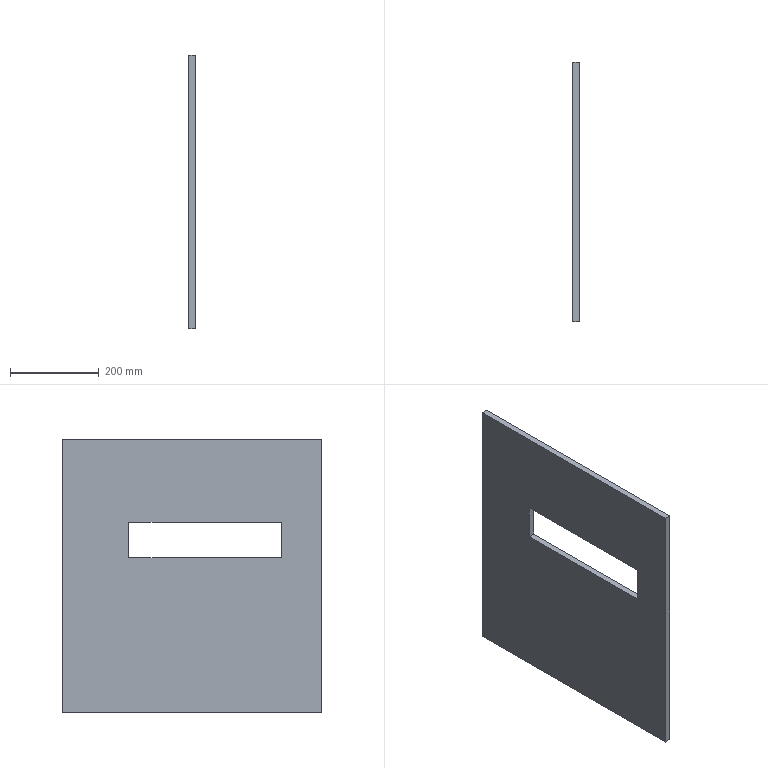Component | NX | PLATE | 1 solid | 10 faces | box 15 x 585 x 618 mm | volume 5008950 mm3 | plane 10
STEP:
#1=CARTESIAN_POINT('',(0.,0.,0.));
#2=DIRECTION('',(0.,0.,1.));
#3=DIRECTION('',(1.,0.,0.));
#4=AXIS2_PLACEMENT_3D('',#1,#2,#3);
#5=CARTESIAN_POINT('',(1548.254,590.,470.));
#6=VERTEX_POINT('',#5);
#7=CARTESIAN_POINT('',(1548.254,935.,470.));
#8=VERTEX_POINT('',#7);
#9=CARTESIAN_POINT('',(1548.254,935.,470.));
#10=DIRECTION('',(0.,1.,0.));
#11=VECTOR('',#10,1.);
#12=LINE('',#9,#11);
#13=CARTESIAN_POINT('',(1533.254,935.,470.));
#14=DIRECTION('',(0.,0.,1.));
#15=DIRECTION('',(0.,-1.,0.));
#16=AXIS2_PLACEMENT_3D('',#13,#14,#15);
#17=PLANE('',#16);
#18=CARTESIAN_POINT('',(0.,15.));
#19=DIRECTION('',(-1.,0.));
#20=VECTOR('',#19,1.);
#21=LINE('',#18,#20);
#22=(GEOMETRIC_REPRESENTATION_CONTEXT(2)PARAMETRIC_REPRESENTATION_CONTEXT()REPRESENTATION_CONTEXT('',''));
#23=DEFINITIONAL_REPRESENTATION('',(#21),#22);
#24=PCURVE('',#17,#23);
#25=CARTESIAN_POINT('',(1548.254,1295.392,39.213));
#26=DIRECTION('',(1.,0.,0.));
#27=DIRECTION('',(0.,1.,0.));
#28=AXIS2_PLACEMENT_3D('',#25,#26,#27);
#29=PLANE('',#28);
#30=CARTESIAN_POINT('',(-360.392,430.787));
#31=DIRECTION('',(1.,0.));
#32=VECTOR('',#31,1.);
#33=LINE('',#30,#32);
#34=(GEOMETRIC_REPRESENTATION_CONTEXT(2)PARAMETRIC_REPRESENTATION_CONTEXT()REPRESENTATION_CONTEXT('',''));
#35=DEFINITIONAL_REPRESENTATION('',(#33),#34);
#36=PCURVE('',#29,#35);
#37=SURFACE_CURVE('',#12,(#24,#36),.PCURVE_S1.);
#38=EDGE_CURVE('',#6,#8,#37,.T.);
#39=ORIENTED_EDGE('',*,*,#38,.T.);
#40=CARTESIAN_POINT('',(1533.254,935.,470.));
#41=VERTEX_POINT('',#40);
#42=CARTESIAN_POINT('',(1533.254,935.,470.));
#43=DIRECTION('',(-1.,0.,0.));
#44=VECTOR('',#43,1.);
#45=LINE('',#42,#44);
#46=CARTESIAN_POINT('',(0.,0.));
#47=DIRECTION('',(0.,-1.));
#48=VECTOR('',#47,1.);
#49=LINE('',#46,#48);
#50=(GEOMETRIC_REPRESENTATION_CONTEXT(2)PARAMETRIC_REPRESENTATION_CONTEXT()REPRESENTATION_CONTEXT('',''));
#51=DEFINITIONAL_REPRESENTATION('',(#49),#50);
#52=PCURVE('',#17,#51);
#53=CARTESIAN_POINT('',(1533.254,935.,550.));
#54=DIRECTION('',(0.,-1.,0.));
#55=DIRECTION('',(1.,0.,0.));
#56=AXIS2_PLACEMENT_3D('',#53,#54,#55);
#57=PLANE('',#56);
#58=CARTESIAN_POINT('',(0.,-80.));
#59=DIRECTION('',(-1.,0.));
#60=VECTOR('',#59,1.);
#61=LINE('',#58,#60);
#62=(GEOMETRIC_REPRESENTATION_CONTEXT(2)PARAMETRIC_REPRESENTATION_CONTEXT()REPRESENTATION_CONTEXT('',''));
#63=DEFINITIONAL_REPRESENTATION('',(#61),#62);
#64=PCURVE('',#57,#63);
#65=SURFACE_CURVE('',#45,(#52,#64),.PCURVE_S1.);
#66=EDGE_CURVE('',#8,#41,#65,.T.);
#67=ORIENTED_EDGE('',*,*,#66,.T.);
#68=CARTESIAN_POINT('',(1533.254,590.,470.));
#69=VERTEX_POINT('',#68);
#70=CARTESIAN_POINT('',(1533.254,935.,470.));
#71=DIRECTION('',(0.,1.,0.));
#72=VECTOR('',#71,1.);
#73=LINE('',#70,#72);
#74=CARTESIAN_POINT('',(0.,0.));
#75=DIRECTION('',(-1.,0.));
#76=VECTOR('',#75,1.);
#77=LINE('',#74,#76);
#78=(GEOMETRIC_REPRESENTATION_CONTEXT(2)PARAMETRIC_REPRESENTATION_CONTEXT()REPRESENTATION_CONTEXT('',''));
#79=DEFINITIONAL_REPRESENTATION('',(#77),#78);
#80=PCURVE('',#17,#79);
#81=CARTESIAN_POINT('',(1533.254,1295.392,39.213));
#82=DIRECTION('',(1.,0.,0.));
#83=DIRECTION('',(0.,1.,0.));
#84=AXIS2_PLACEMENT_3D('',#81,#82,#83);
#85=PLANE('',#84);
#86=CARTESIAN_POINT('',(-360.392,430.787));
#87=DIRECTION('',(1.,0.));
#88=VECTOR('',#87,1.);
#89=LINE('',#86,#88);
#90=(GEOMETRIC_REPRESENTATION_CONTEXT(2)PARAMETRIC_REPRESENTATION_CONTEXT()REPRESENTATION_CONTEXT('',''));
#91=DEFINITIONAL_REPRESENTATION('',(#89),#90);
#92=PCURVE('',#85,#91);
#93=SURFACE_CURVE('',#73,(#80,#92),.PCURVE_S1.);
#94=EDGE_CURVE('',#69,#41,#93,.T.);
#95=ORIENTED_EDGE('',*,*,#94,.F.);
#96=CARTESIAN_POINT('',(1533.254,590.,470.));
#97=DIRECTION('',(-1.,0.,0.));
#98=VECTOR('',#97,1.);
#99=LINE('',#96,#98);
#100=CARTESIAN_POINT('',(345.,0.));
#101=DIRECTION('',(0.,-1.));
#102=VECTOR('',#101,1.);
#103=LINE('',#100,#102);
#104=(GEOMETRIC_REPRESENTATION_CONTEXT(2)PARAMETRIC_REPRESENTATION_CONTEXT()REPRESENTATION_CONTEXT('',''));
#105=DEFINITIONAL_REPRESENTATION('',(#103),#104);
#106=PCURVE('',#17,#105);
#107=CARTESIAN_POINT('',(1533.254,590.,470.));
#108=DIRECTION('',(0.,1.,0.));
#109=DIRECTION('',(-1.,0.,0.));
#110=AXIS2_PLACEMENT_3D('',#107,#108,#109);
#111=PLANE('',#110);
#112=CARTESIAN_POINT('',(0.,0.));
#113=DIRECTION('',(1.,0.));
#114=VECTOR('',#113,1.);
#115=LINE('',#112,#114);
#116=(GEOMETRIC_REPRESENTATION_CONTEXT(2)PARAMETRIC_REPRESENTATION_CONTEXT()REPRESENTATION_CONTEXT('',''));
#117=DEFINITIONAL_REPRESENTATION('',(#115),#116);
#118=PCURVE('',#111,#117);
#119=SURFACE_CURVE('',#99,(#106,#118),.PCURVE_S1.);
#120=EDGE_CURVE('',#6,#69,#119,.T.);
#121=ORIENTED_EDGE('',*,*,#120,.F.);
#122=EDGE_LOOP('',(#39,#67,#95,#121));
#123=FACE_BOUND('',#122,.T.);
#124=ADVANCED_FACE('',(#123),#17,.T.);
#125=CARTESIAN_POINT('',(1548.254,590.,550.));
#126=VERTEX_POINT('',#125);
#127=CARTESIAN_POINT('',(1548.254,590.,470.));
#128=DIRECTION('',(0.,0.,-1.));
#129=VECTOR('',#128,1.);
#130=LINE('',#127,#129);
#131=CARTESIAN_POINT('',(-15.,0.));
#132=DIRECTION('',(0.,-1.));
#133=VECTOR('',#132,1.);
#134=LINE('',#131,#133);
#135=(GEOMETRIC_REPRESENTATION_CONTEXT(2)PARAMETRIC_REPRESENTATION_CONTEXT()REPRESENTATION_CONTEXT('',''));
#136=DEFINITIONAL_REPRESENTATION('',(#134),#135);
#137=PCURVE('',#111,#136);
#138=CARTESIAN_POINT('',(-705.392,430.787));
#139=DIRECTION('',(0.,-1.));
#140=VECTOR('',#139,1.);
#141=LINE('',#138,#140);
#142=(GEOMETRIC_REPRESENTATION_CONTEXT(2)PARAMETRIC_REPRESENTATION_CONTEXT()REPRESENTATION_CONTEXT('',''));
#143=DEFINITIONAL_REPRESENTATION('',(#141),#142);
#144=PCURVE('',#29,#143);
#145=SURFACE_CURVE('',#130,(#137,#144),.PCURVE_S1.);
#146=EDGE_CURVE('',#126,#6,#145,.T.);
#147=ORIENTED_EDGE('',*,*,#146,.T.);
#148=ORIENTED_EDGE('',*,*,#120,.T.);
#149=CARTESIAN_POINT('',(1533.254,590.,550.));
#150=VERTEX_POINT('',#149);
#151=CARTESIAN_POINT('',(1533.254,590.,470.));
#152=DIRECTION('',(0.,0.,-1.));
#153=VECTOR('',#152,1.);
#154=LINE('',#151,#153);
#155=CARTESIAN_POINT('',(0.,0.));
#156=DIRECTION('',(0.,-1.));
#157=VECTOR('',#156,1.);
#158=LINE('',#155,#157);
#159=(GEOMETRIC_REPRESENTATION_CONTEXT(2)PARAMETRIC_REPRESENTATION_CONTEXT()REPRESENTATION_CONTEXT('',''));
#160=DEFINITIONAL_REPRESENTATION('',(#158),#159);
#161=PCURVE('',#111,#160);
#162=CARTESIAN_POINT('',(-705.392,430.787));
#163=DIRECTION('',(0.,-1.));
#164=VECTOR('',#163,1.);
#165=LINE('',#162,#164);
#166=(GEOMETRIC_REPRESENTATION_CONTEXT(2)PARAMETRIC_REPRESENTATION_CONTEXT()REPRESENTATION_CONTEXT('',''));
#167=DEFINITIONAL_REPRESENTATION('',(#165),#166);
#168=PCURVE('',#85,#167);
#169=SURFACE_CURVE('',#154,(#161,#168),.PCURVE_S1.);
#170=EDGE_CURVE('',#150,#69,#169,.T.);
#171=ORIENTED_EDGE('',*,*,#170,.F.);
#172=CARTESIAN_POINT('',(1533.254,590.,550.));
#173=DIRECTION('',(-1.,0.,0.));
#174=VECTOR('',#173,1.);
#175=LINE('',#172,#174);
#176=CARTESIAN_POINT('',(0.,80.));
#177=DIRECTION('',(1.,0.));
#178=VECTOR('',#177,1.);
#179=LINE('',#176,#178);
#180=(GEOMETRIC_REPRESENTATION_CONTEXT(2)PARAMETRIC_REPRESENTATION_CONTEXT()REPRESENTATION_CONTEXT('',''));
#181=DEFINITIONAL_REPRESENTATION('',(#179),#180);
#182=PCURVE('',#111,#181);
#183=CARTESIAN_POINT('',(1533.254,590.,550.));
#184=DIRECTION('',(0.,0.,-1.));
#185=DIRECTION('',(0.,1.,0.));
#186=AXIS2_PLACEMENT_3D('',#183,#184,#185);
#187=PLANE('',#186);
#188=CARTESIAN_POINT('',(0.,0.));
#189=DIRECTION('',(0.,-1.));
#190=VECTOR('',#189,1.);
#191=LINE('',#188,#190);
#192=(GEOMETRIC_REPRESENTATION_CONTEXT(2)PARAMETRIC_REPRESENTATION_CONTEXT()REPRESENTATION_CONTEXT('',''));
#193=DEFINITIONAL_REPRESENTATION('',(#191),#192);
#194=PCURVE('',#187,#193);
#195=SURFACE_CURVE('',#175,(#182,#194),.PCURVE_S1.);
#196=EDGE_CURVE('',#126,#150,#195,.T.);
#197=ORIENTED_EDGE('',*,*,#196,.F.);
#198=EDGE_LOOP('',(#147,#148,#171,#197));
#199=FACE_BOUND('',#198,.T.);
#200=ADVANCED_FACE('',(#199),#111,.T.);
#201=CARTESIAN_POINT('',(1548.254,935.,550.));
#202=VERTEX_POINT('',#201);
#203=CARTESIAN_POINT('',(1548.254,590.,550.));
#204=DIRECTION('',(0.,-1.,0.));
#205=VECTOR('',#204,1.);
#206=LINE('',#203,#205);
#207=CARTESIAN_POINT('',(0.,15.));
#208=DIRECTION('',(-1.,0.));
#209=VECTOR('',#208,1.);
#210=LINE('',#207,#209);
#211=(GEOMETRIC_REPRESENTATION_CONTEXT(2)PARAMETRIC_REPRESENTATION_CONTEXT()REPRESENTATION_CONTEXT('',''));
#212=DEFINITIONAL_REPRESENTATION('',(#210),#211);
#213=PCURVE('',#187,#212);
#214=CARTESIAN_POINT('',(-705.392,510.787));
#215=DIRECTION('',(-1.,0.));
#216=VECTOR('',#215,1.);
#217=LINE('',#214,#216);
#218=(GEOMETRIC_REPRESENTATION_CONTEXT(2)PARAMETRIC_REPRESENTATION_CONTEXT()REPRESENTATION_CONTEXT('',''));
#219=DEFINITIONAL_REPRESENTATION('',(#217),#218);
#220=PCURVE('',#29,#219);
#221=SURFACE_CURVE('',#206,(#213,#220),.PCURVE_S1.);
#222=EDGE_CURVE('',#202,#126,#221,.T.);
#223=ORIENTED_EDGE('',*,*,#222,.T.);
#224=ORIENTED_EDGE('',*,*,#196,.T.);
#225=CARTESIAN_POINT('',(1533.254,935.,550.));
#226=VERTEX_POINT('',#225);
#227=CARTESIAN_POINT('',(1533.254,590.,550.));
#228=DIRECTION('',(0.,-1.,0.));
#229=VECTOR('',#228,1.);
#230=LINE('',#227,#229);
#231=CARTESIAN_POINT('',(0.,0.));
#232=DIRECTION('',(-1.,0.));
#233=VECTOR('',#232,1.);
#234=LINE('',#231,#233);
#235=(GEOMETRIC_REPRESENTATION_CONTEXT(2)PARAMETRIC_REPRESENTATION_CONTEXT()REPRESENTATION_CONTEXT('',''));
#236=DEFINITIONAL_REPRESENTATION('',(#234),#235);
#237=PCURVE('',#187,#236);
#238=CARTESIAN_POINT('',(-705.392,510.787));
#239=DIRECTION('',(-1.,0.));
#240=VECTOR('',#239,1.);
#241=LINE('',#238,#240);
#242=(GEOMETRIC_REPRESENTATION_CONTEXT(2)PARAMETRIC_REPRESENTATION_CONTEXT()REPRESENTATION_CONTEXT('',''));
#243=DEFINITIONAL_REPRESENTATION('',(#241),#242);
#244=PCURVE('',#85,#243);
#245=SURFACE_CURVE('',#230,(#237,#244),.PCURVE_S1.);
#246=EDGE_CURVE('',#226,#150,#245,.T.);
#247=ORIENTED_EDGE('',*,*,#246,.F.);
#248=CARTESIAN_POINT('',(1533.254,935.,550.));
#249=DIRECTION('',(-1.,0.,0.));
#250=VECTOR('',#249,1.);
#251=LINE('',#248,#250);
#252=CARTESIAN_POINT('',(345.,0.));
#253=DIRECTION('',(0.,-1.));
#254=VECTOR('',#253,1.);
#255=LINE('',#252,#254);
#256=(GEOMETRIC_REPRESENTATION_CONTEXT(2)PARAMETRIC_REPRESENTATION_CONTEXT()REPRESENTATION_CONTEXT('',''));
#257=DEFINITIONAL_REPRESENTATION('',(#255),#256);
#258=PCURVE('',#187,#257);
#259=CARTESIAN_POINT('',(0.,0.));
#260=DIRECTION('',(-1.,0.));
#261=VECTOR('',#260,1.);
#262=LINE('',#259,#261);
#263=(GEOMETRIC_REPRESENTATION_CONTEXT(2)PARAMETRIC_REPRESENTATION_CONTEXT()REPRESENTATION_CONTEXT('',''));
#264=DEFINITIONAL_REPRESENTATION('',(#262),#263);
#265=PCURVE('',#57,#264);
#266=SURFACE_CURVE('',#251,(#258,#265),.PCURVE_S1.);
#267=EDGE_CURVE('',#202,#226,#266,.T.);
#268=ORIENTED_EDGE('',*,*,#267,.F.);
#269=EDGE_LOOP('',(#223,#224,#247,#268));
#270=FACE_BOUND('',#269,.T.);
#271=ADVANCED_FACE('',(#270),#187,.T.);
#272=CARTESIAN_POINT('',(1548.254,1085.,120.));
#273=VERTEX_POINT('',#272);
#274=CARTESIAN_POINT('',(1548.254,500.,120.));
#275=VERTEX_POINT('',#274);
#276=CARTESIAN_POINT('',(1548.254,500.,120.));
#277=DIRECTION('',(0.,-1.,0.));
#278=VECTOR('',#277,1.);
#279=LINE('',#276,#278);
#280=CARTESIAN_POINT('',(1533.254,500.,120.));
#281=DIRECTION('',(0.,0.,-1.));
#282=DIRECTION('',(0.,1.,0.));
#283=AXIS2_PLACEMENT_3D('',#280,#281,#282);
#284=PLANE('',#283);
#285=CARTESIAN_POINT('',(0.,15.));
#286=DIRECTION('',(-1.,0.));
#287=VECTOR('',#286,1.);
#288=LINE('',#285,#287);
#289=(GEOMETRIC_REPRESENTATION_CONTEXT(2)PARAMETRIC_REPRESENTATION_CONTEXT()REPRESENTATION_CONTEXT('',''));
#290=DEFINITIONAL_REPRESENTATION('',(#288),#289);
#291=PCURVE('',#284,#290);
#292=CARTESIAN_POINT('',(-795.392,80.787));
#293=DIRECTION('',(-1.,0.));
#294=VECTOR('',#293,1.);
#295=LINE('',#292,#294);
#296=(GEOMETRIC_REPRESENTATION_CONTEXT(2)PARAMETRIC_REPRESENTATION_CONTEXT()REPRESENTATION_CONTEXT('',''));
#297=DEFINITIONAL_REPRESENTATION('',(#295),#296);
#298=PCURVE('',#29,#297);
#299=SURFACE_CURVE('',#279,(#291,#298),.PCURVE_S1.);
#300=EDGE_CURVE('',#273,#275,#299,.T.);
#301=ORIENTED_EDGE('',*,*,#300,.T.);
#302=CARTESIAN_POINT('',(1533.254,500.,120.));
#303=VERTEX_POINT('',#302);
#304=CARTESIAN_POINT('',(1533.254,500.,120.));
#305=DIRECTION('',(-1.,0.,0.));
#306=VECTOR('',#305,1.);
#307=LINE('',#304,#306);
#308=CARTESIAN_POINT('',(0.,0.));
#309=DIRECTION('',(0.,-1.));
#310=VECTOR('',#309,1.);
#311=LINE('',#308,#310);
#312=(GEOMETRIC_REPRESENTATION_CONTEXT(2)PARAMETRIC_REPRESENTATION_CONTEXT()REPRESENTATION_CONTEXT('',''));
#313=DEFINITIONAL_REPRESENTATION('',(#311),#312);
#314=PCURVE('',#284,#313);
#315=CARTESIAN_POINT('',(1533.254,500.,738.));
#316=DIRECTION('',(0.,-1.,0.));
#317=DIRECTION('',(1.,0.,0.));
#318=AXIS2_PLACEMENT_3D('',#315,#316,#317);
#319=PLANE('',#318);
#320=CARTESIAN_POINT('',(0.,-618.));
#321=DIRECTION('',(-1.,0.));
#322=VECTOR('',#321,1.);
#323=LINE('',#320,#322);
#324=(GEOMETRIC_REPRESENTATION_CONTEXT(2)PARAMETRIC_REPRESENTATION_CONTEXT()REPRESENTATION_CONTEXT('',''));
#325=DEFINITIONAL_REPRESENTATION('',(#323),#324);
#326=PCURVE('',#319,#325);
#327=SURFACE_CURVE('',#307,(#314,#326),.PCURVE_S1.);
#328=EDGE_CURVE('',#275,#303,#327,.T.);
#329=ORIENTED_EDGE('',*,*,#328,.T.);
#330=CARTESIAN_POINT('',(1533.254,1085.,120.));
#331=VERTEX_POINT('',#330);
#332=CARTESIAN_POINT('',(1533.254,500.,120.));
#333=DIRECTION('',(0.,-1.,0.));
#334=VECTOR('',#333,1.);
#335=LINE('',#332,#334);
#336=CARTESIAN_POINT('',(0.,0.));
#337=DIRECTION('',(-1.,0.));
#338=VECTOR('',#337,1.);
#339=LINE('',#336,#338);
#340=(GEOMETRIC_REPRESENTATION_CONTEXT(2)PARAMETRIC_REPRESENTATION_CONTEXT()REPRESENTATION_CONTEXT('',''));
#341=DEFINITIONAL_REPRESENTATION('',(#339),#340);
#342=PCURVE('',#284,#341);
#343=CARTESIAN_POINT('',(-795.392,80.787));
#344=DIRECTION('',(-1.,0.));
#345=VECTOR('',#344,1.);
#346=LINE('',#343,#345);
#347=(GEOMETRIC_REPRESENTATION_CONTEXT(2)PARAMETRIC_REPRESENTATION_CONTEXT()REPRESENTATION_CONTEXT('',''));
#348=DEFINITIONAL_REPRESENTATION('',(#346),#347);
#349=PCURVE('',#85,#348);
#350=SURFACE_CURVE('',#335,(#342,#349),.PCURVE_S1.);
#351=EDGE_CURVE('',#331,#303,#350,.T.);
#352=ORIENTED_EDGE('',*,*,#351,.F.);
#353=CARTESIAN_POINT('',(1533.254,1085.,120.));
#354=DIRECTION('',(-1.,0.,0.));
#355=VECTOR('',#354,1.);
#356=LINE('',#353,#355);
#357=CARTESIAN_POINT('',(585.,0.));
#358=DIRECTION('',(0.,-1.));
#359=VECTOR('',#358,1.);
#360=LINE('',#357,#359);
#361=(GEOMETRIC_REPRESENTATION_CONTEXT(2)PARAMETRIC_REPRESENTATION_CONTEXT()REPRESENTATION_CONTEXT('',''));
#362=DEFINITIONAL_REPRESENTATION('',(#360),#361);
#363=PCURVE('',#284,#362);
#364=CARTESIAN_POINT('',(1533.254,1085.,120.));
#365=DIRECTION('',(0.,1.,0.));
#366=DIRECTION('',(-1.,0.,0.));
#367=AXIS2_PLACEMENT_3D('',#364,#365,#366);
#368=PLANE('',#367);
#369=CARTESIAN_POINT('',(0.,0.));
#370=DIRECTION('',(1.,0.));
#371=VECTOR('',#370,1.);
#372=LINE('',#369,#371);
#373=(GEOMETRIC_REPRESENTATION_CONTEXT(2)PARAMETRIC_REPRESENTATION_CONTEXT()REPRESENTATION_CONTEXT('',''));
#374=DEFINITIONAL_REPRESENTATION('',(#372),#373);
#375=PCURVE('',#368,#374);
#376=SURFACE_CURVE('',#356,(#363,#375),.PCURVE_S1.);
#377=EDGE_CURVE('',#273,#331,#376,.T.);
#378=ORIENTED_EDGE('',*,*,#377,.F.);
#379=EDGE_LOOP('',(#301,#329,#352,#378));
#380=FACE_BOUND('',#379,.T.);
#381=ADVANCED_FACE('',(#380),#284,.T.);
#382=CARTESIAN_POINT('',(1548.254,1085.,738.));
#383=VERTEX_POINT('',#382);
#384=CARTESIAN_POINT('',(1548.254,1085.,120.));
#385=DIRECTION('',(0.,0.,-1.));
#386=VECTOR('',#385,1.);
#387=LINE('',#384,#386);
#388=CARTESIAN_POINT('',(-15.,0.));
#389=DIRECTION('',(0.,-1.));
#390=VECTOR('',#389,1.);
#391=LINE('',#388,#390);
#392=(GEOMETRIC_REPRESENTATION_CONTEXT(2)PARAMETRIC_REPRESENTATION_CONTEXT()REPRESENTATION_CONTEXT('',''));
#393=DEFINITIONAL_REPRESENTATION('',(#391),#392);
#394=PCURVE('',#368,#393);
#395=CARTESIAN_POINT('',(-210.392,80.787));
#396=DIRECTION('',(0.,-1.));
#397=VECTOR('',#396,1.);
#398=LINE('',#395,#397);
#399=(GEOMETRIC_REPRESENTATION_CONTEXT(2)PARAMETRIC_REPRESENTATION_CONTEXT()REPRESENTATION_CONTEXT('',''));
#400=DEFINITIONAL_REPRESENTATION('',(#398),#399);
#401=PCURVE('',#29,#400);
#402=SURFACE_CURVE('',#387,(#394,#401),.PCURVE_S1.);
#403=EDGE_CURVE('',#383,#273,#402,.T.);
#404=ORIENTED_EDGE('',*,*,#403,.T.);
#405=ORIENTED_EDGE('',*,*,#377,.T.);
#406=CARTESIAN_POINT('',(1533.254,1085.,738.));
#407=VERTEX_POINT('',#406);
#408=CARTESIAN_POINT('',(1533.254,1085.,120.));
#409=DIRECTION('',(0.,0.,-1.));
#410=VECTOR('',#409,1.);
#411=LINE('',#408,#410);
#412=CARTESIAN_POINT('',(0.,0.));
#413=DIRECTION('',(0.,-1.));
#414=VECTOR('',#413,1.);
#415=LINE('',#412,#414);
#416=(GEOMETRIC_REPRESENTATION_CONTEXT(2)PARAMETRIC_REPRESENTATION_CONTEXT()REPRESENTATION_CONTEXT('',''));
#417=DEFINITIONAL_REPRESENTATION('',(#415),#416);
#418=PCURVE('',#368,#417);
#419=CARTESIAN_POINT('',(-210.392,80.787));
#420=DIRECTION('',(0.,-1.));
#421=VECTOR('',#420,1.);
#422=LINE('',#419,#421);
#423=(GEOMETRIC_REPRESENTATION_CONTEXT(2)PARAMETRIC_REPRESENTATION_CONTEXT()REPRESENTATION_CONTEXT('',''));
#424=DEFINITIONAL_REPRESENTATION('',(#422),#423);
#425=PCURVE('',#85,#424);
#426=SURFACE_CURVE('',#411,(#418,#425),.PCURVE_S1.);
#427=EDGE_CURVE('',#407,#331,#426,.T.);
#428=ORIENTED_EDGE('',*,*,#427,.F.);
#429=CARTESIAN_POINT('',(1533.254,1085.,738.));
#430=DIRECTION('',(-1.,0.,0.));
#431=VECTOR('',#430,1.);
#432=LINE('',#429,#431);
#433=CARTESIAN_POINT('',(0.,618.));
#434=DIRECTION('',(1.,0.));
#435=VECTOR('',#434,1.);
#436=LINE('',#433,#435);
#437=(GEOMETRIC_REPRESENTATION_CONTEXT(2)PARAMETRIC_REPRESENTATION_CONTEXT()REPRESENTATION_CONTEXT('',''));
#438=DEFINITIONAL_REPRESENTATION('',(#436),#437);
#439=PCURVE('',#368,#438);
#440=CARTESIAN_POINT('',(1533.254,1085.,738.));
#441=DIRECTION('',(0.,0.,1.));
#442=DIRECTION('',(0.,-1.,0.));
#443=AXIS2_PLACEMENT_3D('',#440,#441,#442);
#444=PLANE('',#443);
#445=CARTESIAN_POINT('',(0.,0.));
#446=DIRECTION('',(0.,-1.));
#447=VECTOR('',#446,1.);
#448=LINE('',#445,#447);
#449=(GEOMETRIC_REPRESENTATION_CONTEXT(2)PARAMETRIC_REPRESENTATION_CONTEXT()REPRESENTATION_CONTEXT('',''));
#450=DEFINITIONAL_REPRESENTATION('',(#448),#449);
#451=PCURVE('',#444,#450);
#452=SURFACE_CURVE('',#432,(#439,#451),.PCURVE_S1.);
#453=EDGE_CURVE('',#383,#407,#452,.T.);
#454=ORIENTED_EDGE('',*,*,#453,.F.);
#455=EDGE_LOOP('',(#404,#405,#428,#454));
#456=FACE_BOUND('',#455,.T.);
#457=ADVANCED_FACE('',(#456),#368,.T.);
#458=CARTESIAN_POINT('',(1548.254,500.,738.));
#459=VERTEX_POINT('',#458);
#460=CARTESIAN_POINT('',(1548.254,1085.,738.));
#461=DIRECTION('',(0.,1.,0.));
#462=VECTOR('',#461,1.);
#463=LINE('',#460,#462);
#464=CARTESIAN_POINT('',(0.,15.));
#465=DIRECTION('',(-1.,0.));
#466=VECTOR('',#465,1.);
#467=LINE('',#464,#466);
#468=(GEOMETRIC_REPRESENTATION_CONTEXT(2)PARAMETRIC_REPRESENTATION_CONTEXT()REPRESENTATION_CONTEXT('',''));
#469=DEFINITIONAL_REPRESENTATION('',(#467),#468);
#470=PCURVE('',#444,#469);
#471=CARTESIAN_POINT('',(-210.392,698.787));
#472=DIRECTION('',(1.,0.));
#473=VECTOR('',#472,1.);
#474=LINE('',#471,#473);
#475=(GEOMETRIC_REPRESENTATION_CONTEXT(2)PARAMETRIC_REPRESENTATION_CONTEXT()REPRESENTATION_CONTEXT('',''));
#476=DEFINITIONAL_REPRESENTATION('',(#474),#475);
#477=PCURVE('',#29,#476);
#478=SURFACE_CURVE('',#463,(#470,#477),.PCURVE_S1.);
#479=EDGE_CURVE('',#459,#383,#478,.T.);
#480=ORIENTED_EDGE('',*,*,#479,.T.);
#481=ORIENTED_EDGE('',*,*,#453,.T.);
#482=CARTESIAN_POINT('',(1533.254,500.,738.));
#483=VERTEX_POINT('',#482);
#484=CARTESIAN_POINT('',(1533.254,1085.,738.));
#485=DIRECTION('',(0.,1.,0.));
#486=VECTOR('',#485,1.);
#487=LINE('',#484,#486);
#488=CARTESIAN_POINT('',(0.,0.));
#489=DIRECTION('',(-1.,0.));
#490=VECTOR('',#489,1.);
#491=LINE('',#488,#490);
#492=(GEOMETRIC_REPRESENTATION_CONTEXT(2)PARAMETRIC_REPRESENTATION_CONTEXT()REPRESENTATION_CONTEXT('',''));
#493=DEFINITIONAL_REPRESENTATION('',(#491),#492);
#494=PCURVE('',#444,#493);
#495=CARTESIAN_POINT('',(-210.392,698.787));
#496=DIRECTION('',(1.,0.));
#497=VECTOR('',#496,1.);
#498=LINE('',#495,#497);
#499=(GEOMETRIC_REPRESENTATION_CONTEXT(2)PARAMETRIC_REPRESENTATION_CONTEXT()REPRESENTATION_CONTEXT('',''));
#500=DEFINITIONAL_REPRESENTATION('',(#498),#499);
#501=PCURVE('',#85,#500);
#502=SURFACE_CURVE('',#487,(#494,#501),.PCURVE_S1.);
#503=EDGE_CURVE('',#483,#407,#502,.T.);
#504=ORIENTED_EDGE('',*,*,#503,.F.);
#505=CARTESIAN_POINT('',(1533.254,500.,738.));
#506=DIRECTION('',(-1.,0.,0.));
#507=VECTOR('',#506,1.);
#508=LINE('',#505,#507);
#509=CARTESIAN_POINT('',(585.,0.));
#510=DIRECTION('',(0.,-1.));
#511=VECTOR('',#510,1.);
#512=LINE('',#509,#511);
#513=(GEOMETRIC_REPRESENTATION_CONTEXT(2)PARAMETRIC_REPRESENTATION_CONTEXT()REPRESENTATION_CONTEXT('',''));
#514=DEFINITIONAL_REPRESENTATION('',(#512),#513);
#515=PCURVE('',#444,#514);
#516=CARTESIAN_POINT('',(0.,0.));
#517=DIRECTION('',(-1.,0.));
#518=VECTOR('',#517,1.);
#519=LINE('',#516,#518);
#520=(GEOMETRIC_REPRESENTATION_CONTEXT(2)PARAMETRIC_REPRESENTATION_CONTEXT()REPRESENTATION_CONTEXT('',''));
#521=DEFINITIONAL_REPRESENTATION('',(#519),#520);
#522=PCURVE('',#319,#521);
#523=SURFACE_CURVE('',#508,(#515,#522),.PCURVE_S1.);
#524=EDGE_CURVE('',#459,#483,#523,.T.);
#525=ORIENTED_EDGE('',*,*,#524,.F.);
#526=EDGE_LOOP('',(#480,#481,#504,#525));
#527=FACE_BOUND('',#526,.T.);
#528=ADVANCED_FACE('',(#527),#444,.T.);
#529=CARTESIAN_POINT('',(1548.254,500.,738.));
#530=DIRECTION('',(0.,0.,1.));
#531=VECTOR('',#530,1.);
#532=LINE('',#529,#531);
#533=CARTESIAN_POINT('',(15.,0.));
#534=DIRECTION('',(0.,1.));
#535=VECTOR('',#534,1.);
#536=LINE('',#533,#535);
#537=(GEOMETRIC_REPRESENTATION_CONTEXT(2)PARAMETRIC_REPRESENTATION_CONTEXT()REPRESENTATION_CONTEXT('',''));
#538=DEFINITIONAL_REPRESENTATION('',(#536),#537);
#539=PCURVE('',#319,#538);
#540=CARTESIAN_POINT('',(-795.392,698.787));
#541=DIRECTION('',(0.,1.));
#542=VECTOR('',#541,1.);
#543=LINE('',#540,#542);
#544=(GEOMETRIC_REPRESENTATION_CONTEXT(2)PARAMETRIC_REPRESENTATION_CONTEXT()REPRESENTATION_CONTEXT('',''));
#545=DEFINITIONAL_REPRESENTATION('',(#543),#544);
#546=PCURVE('',#29,#545);
#547=SURFACE_CURVE('',#532,(#539,#546),.PCURVE_S1.);
#548=EDGE_CURVE('',#275,#459,#547,.T.);
#549=ORIENTED_EDGE('',*,*,#548,.T.);
#550=ORIENTED_EDGE('',*,*,#524,.T.);
#551=CARTESIAN_POINT('',(1533.254,500.,738.));
#552=DIRECTION('',(0.,0.,1.));
#553=VECTOR('',#552,1.);
#554=LINE('',#551,#553);
#555=CARTESIAN_POINT('',(0.,0.));
#556=DIRECTION('',(0.,1.));
#557=VECTOR('',#556,1.);
#558=LINE('',#555,#557);
#559=(GEOMETRIC_REPRESENTATION_CONTEXT(2)PARAMETRIC_REPRESENTATION_CONTEXT()REPRESENTATION_CONTEXT('',''));
#560=DEFINITIONAL_REPRESENTATION('',(#558),#559);
#561=PCURVE('',#319,#560);
#562=CARTESIAN_POINT('',(-795.392,698.787));
#563=DIRECTION('',(0.,1.));
#564=VECTOR('',#563,1.);
#565=LINE('',#562,#564);
#566=(GEOMETRIC_REPRESENTATION_CONTEXT(2)PARAMETRIC_REPRESENTATION_CONTEXT()REPRESENTATION_CONTEXT('',''));
#567=DEFINITIONAL_REPRESENTATION('',(#565),#566);
#568=PCURVE('',#85,#567);
#569=SURFACE_CURVE('',#554,(#561,#568),.PCURVE_S1.);
#570=EDGE_CURVE('',#303,#483,#569,.T.);
#571=ORIENTED_EDGE('',*,*,#570,.F.);
#572=ORIENTED_EDGE('',*,*,#328,.F.);
#573=EDGE_LOOP('',(#549,#550,#571,#572));
#574=FACE_BOUND('',#573,.T.);
#575=ADVANCED_FACE('',(#574),#319,.T.);
#576=CARTESIAN_POINT('',(1548.254,935.,550.));
#577=DIRECTION('',(0.,0.,1.));
#578=VECTOR('',#577,1.);
#579=LINE('',#576,#578);
#580=CARTESIAN_POINT('',(15.,0.));
#581=DIRECTION('',(0.,1.));
#582=VECTOR('',#581,1.);
#583=LINE('',#580,#582);
#584=(GEOMETRIC_REPRESENTATION_CONTEXT(2)PARAMETRIC_REPRESENTATION_CONTEXT()REPRESENTATION_CONTEXT('',''));
#585=DEFINITIONAL_REPRESENTATION('',(#583),#584);
#586=PCURVE('',#57,#585);
#587=CARTESIAN_POINT('',(-360.392,510.787));
#588=DIRECTION('',(0.,1.));
#589=VECTOR('',#588,1.);
#590=LINE('',#587,#589);
#591=(GEOMETRIC_REPRESENTATION_CONTEXT(2)PARAMETRIC_REPRESENTATION_CONTEXT()REPRESENTATION_CONTEXT('',''));
#592=DEFINITIONAL_REPRESENTATION('',(#590),#591);
#593=PCURVE('',#29,#592);
#594=SURFACE_CURVE('',#579,(#586,#593),.PCURVE_S1.);
#595=EDGE_CURVE('',#8,#202,#594,.T.);
#596=ORIENTED_EDGE('',*,*,#595,.T.);
#597=ORIENTED_EDGE('',*,*,#267,.T.);
#598=CARTESIAN_POINT('',(1533.254,935.,550.));
#599=DIRECTION('',(0.,0.,1.));
#600=VECTOR('',#599,1.);
#601=LINE('',#598,#600);
#602=CARTESIAN_POINT('',(0.,0.));
#603=DIRECTION('',(0.,1.));
#604=VECTOR('',#603,1.);
#605=LINE('',#602,#604);
#606=(GEOMETRIC_REPRESENTATION_CONTEXT(2)PARAMETRIC_REPRESENTATION_CONTEXT()REPRESENTATION_CONTEXT('',''));
#607=DEFINITIONAL_REPRESENTATION('',(#605),#606);
#608=PCURVE('',#57,#607);
#609=CARTESIAN_POINT('',(-360.392,510.787));
#610=DIRECTION('',(0.,1.));
#611=VECTOR('',#610,1.);
#612=LINE('',#609,#611);
#613=(GEOMETRIC_REPRESENTATION_CONTEXT(2)PARAMETRIC_REPRESENTATION_CONTEXT()REPRESENTATION_CONTEXT('',''));
#614=DEFINITIONAL_REPRESENTATION('',(#612),#613);
#615=PCURVE('',#85,#614);
#616=SURFACE_CURVE('',#601,(#608,#615),.PCURVE_S1.);
#617=EDGE_CURVE('',#41,#226,#616,.T.);
#618=ORIENTED_EDGE('',*,*,#617,.F.);
#619=ORIENTED_EDGE('',*,*,#66,.F.);
#620=EDGE_LOOP('',(#596,#597,#618,#619));
#621=FACE_BOUND('',#620,.T.);
#622=ADVANCED_FACE('',(#621),#57,.T.);
#623=ORIENTED_EDGE('',*,*,#351,.T.);
#624=ORIENTED_EDGE('',*,*,#570,.T.);
#625=ORIENTED_EDGE('',*,*,#503,.T.);
#626=ORIENTED_EDGE('',*,*,#427,.T.);
#627=EDGE_LOOP('',(#623,#624,#625,#626));
#628=FACE_BOUND('',#627,.T.);
#629=ORIENTED_EDGE('',*,*,#94,.T.);
#630=ORIENTED_EDGE('',*,*,#617,.T.);
#631=ORIENTED_EDGE('',*,*,#246,.T.);
#632=ORIENTED_EDGE('',*,*,#170,.T.);
#633=EDGE_LOOP('',(#629,#630,#631,#632));
#634=FACE_BOUND('',#633,.T.);
#635=ADVANCED_FACE('',(#628,#634),#85,.F.);
#636=ORIENTED_EDGE('',*,*,#300,.F.);
#637=ORIENTED_EDGE('',*,*,#403,.F.);
#638=ORIENTED_EDGE('',*,*,#479,.F.);
#639=ORIENTED_EDGE('',*,*,#548,.F.);
#640=EDGE_LOOP('',(#636,#637,#638,#639));
#641=FACE_BOUND('',#640,.T.);
#642=ORIENTED_EDGE('',*,*,#38,.F.);
#643=ORIENTED_EDGE('',*,*,#146,.F.);
#644=ORIENTED_EDGE('',*,*,#222,.F.);
#645=ORIENTED_EDGE('',*,*,#595,.F.);
#646=EDGE_LOOP('',(#642,#643,#644,#645));
#647=FACE_BOUND('',#646,.T.);
#648=ADVANCED_FACE('',(#641,#647),#29,.T.);
#649=CLOSED_SHELL('',(#124,#200,#271,#381,#457,#528,#575,#622,#635,#648));
#650=MANIFOLD_SOLID_BREP('',#649);
#651=(LENGTH_UNIT()NAMED_UNIT(*)SI_UNIT(.MILLI.,.METRE.));
#652=UNCERTAINTY_MEASURE_WITH_UNIT(LENGTH_MEASURE(0.0000001),#651,'','');
#653=(NAMED_UNIT(*)PLANE_ANGLE_UNIT()SI_UNIT($,.RADIAN.));
#654=(NAMED_UNIT(*)SI_UNIT($,.STERADIAN.)SOLID_ANGLE_UNIT());
#655=(GEOMETRIC_REPRESENTATION_CONTEXT(3)GLOBAL_UNCERTAINTY_ASSIGNED_CONTEXT((#652))GLOBAL_UNIT_ASSIGNED_CONTEXT((#651,#653,#654))REPRESENTATION_CONTEXT('',''));
#656=ADVANCED_BREP_SHAPE_REPRESENTATION('',(#4,#650),#655);